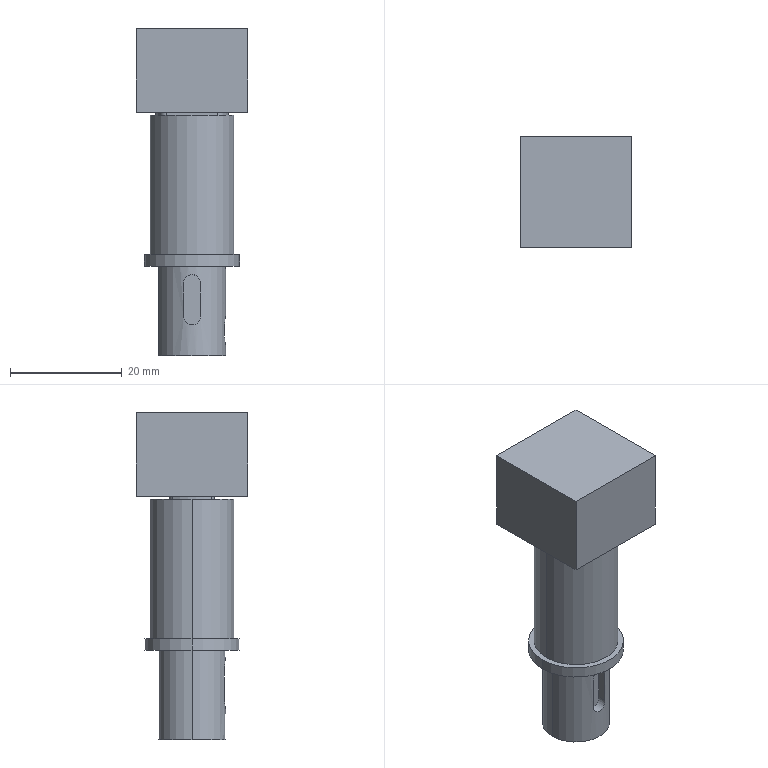CAM job | Mastercam | mm | 18 operations | part box 20 x 20 x 58.5
1. Contour (2D) | 12 - 10 平铣刀
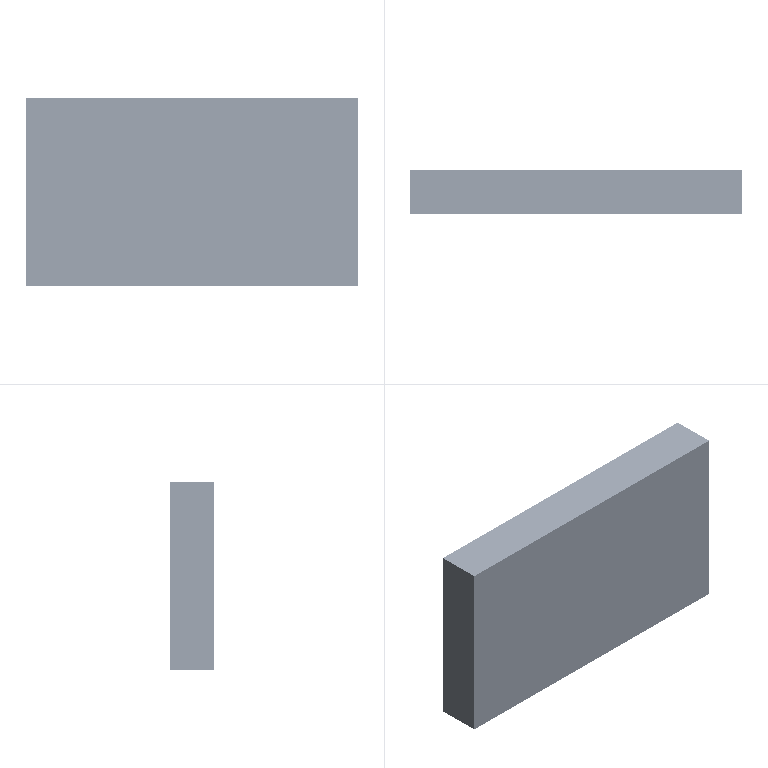2. Contour (2D) | 10 - 12 平铣刀
3. Contour (2D) | 10 - 12 平铣刀
4. Contour (2D chamfer) | 5 - 4 倒角刀
5. Facing | 20 - 63 平铣刀
6. Contour (Ramp) | 8 - 8 平铣刀
7. Contour (Ramp) | 8 - 8 平铣刀
8. Contour (Ramp) | 4 - 4 平铣刀
9. Contour (Remachining) | 2 - 2 平铣刀
10. Contour (Ramp) | 2 - 2 平铣刀
11. 2D High Speed (2D Area Mill) | 2 - 2 平铣刀
12. Contour (2D chamfer) | 5 - 4 倒角刀
13. Contour (Ramp) | 2 - 2 平铣刀
14. Contour (Ramp) | 2 - 2 平铣刀
15. Contour (2D) | 14 - 2 平铣刀
16. Contour (Ramp) | 15 - 6 平铣刀
17. Contour (2D) | 6 - 6 平铣刀
18. Contour (2D chamfer) | 5 - 4 倒角刀